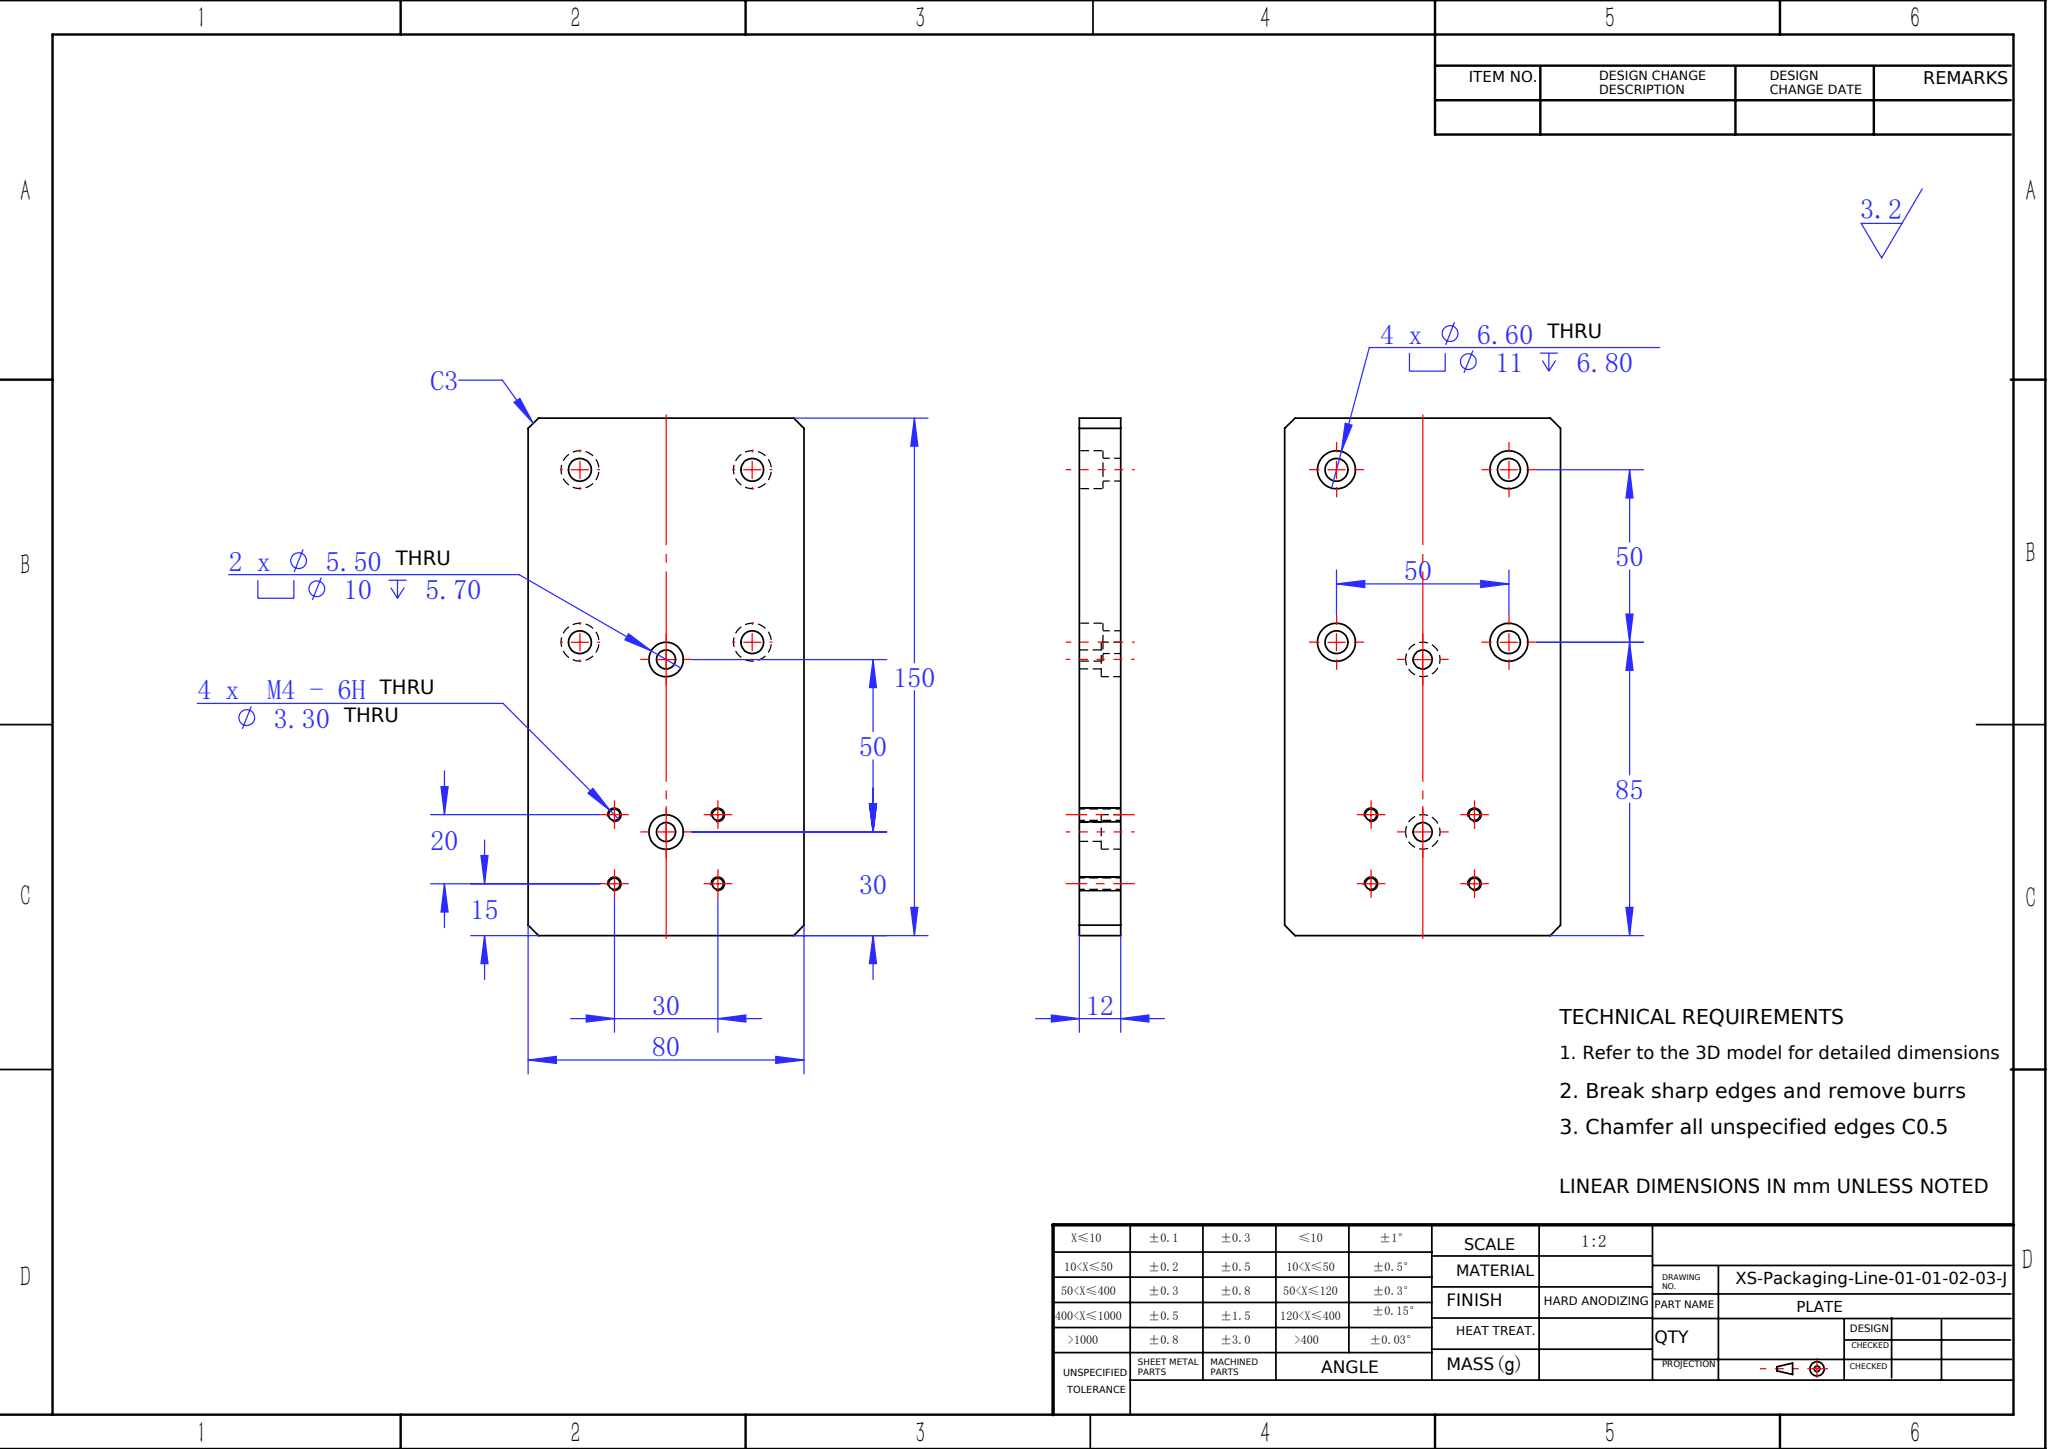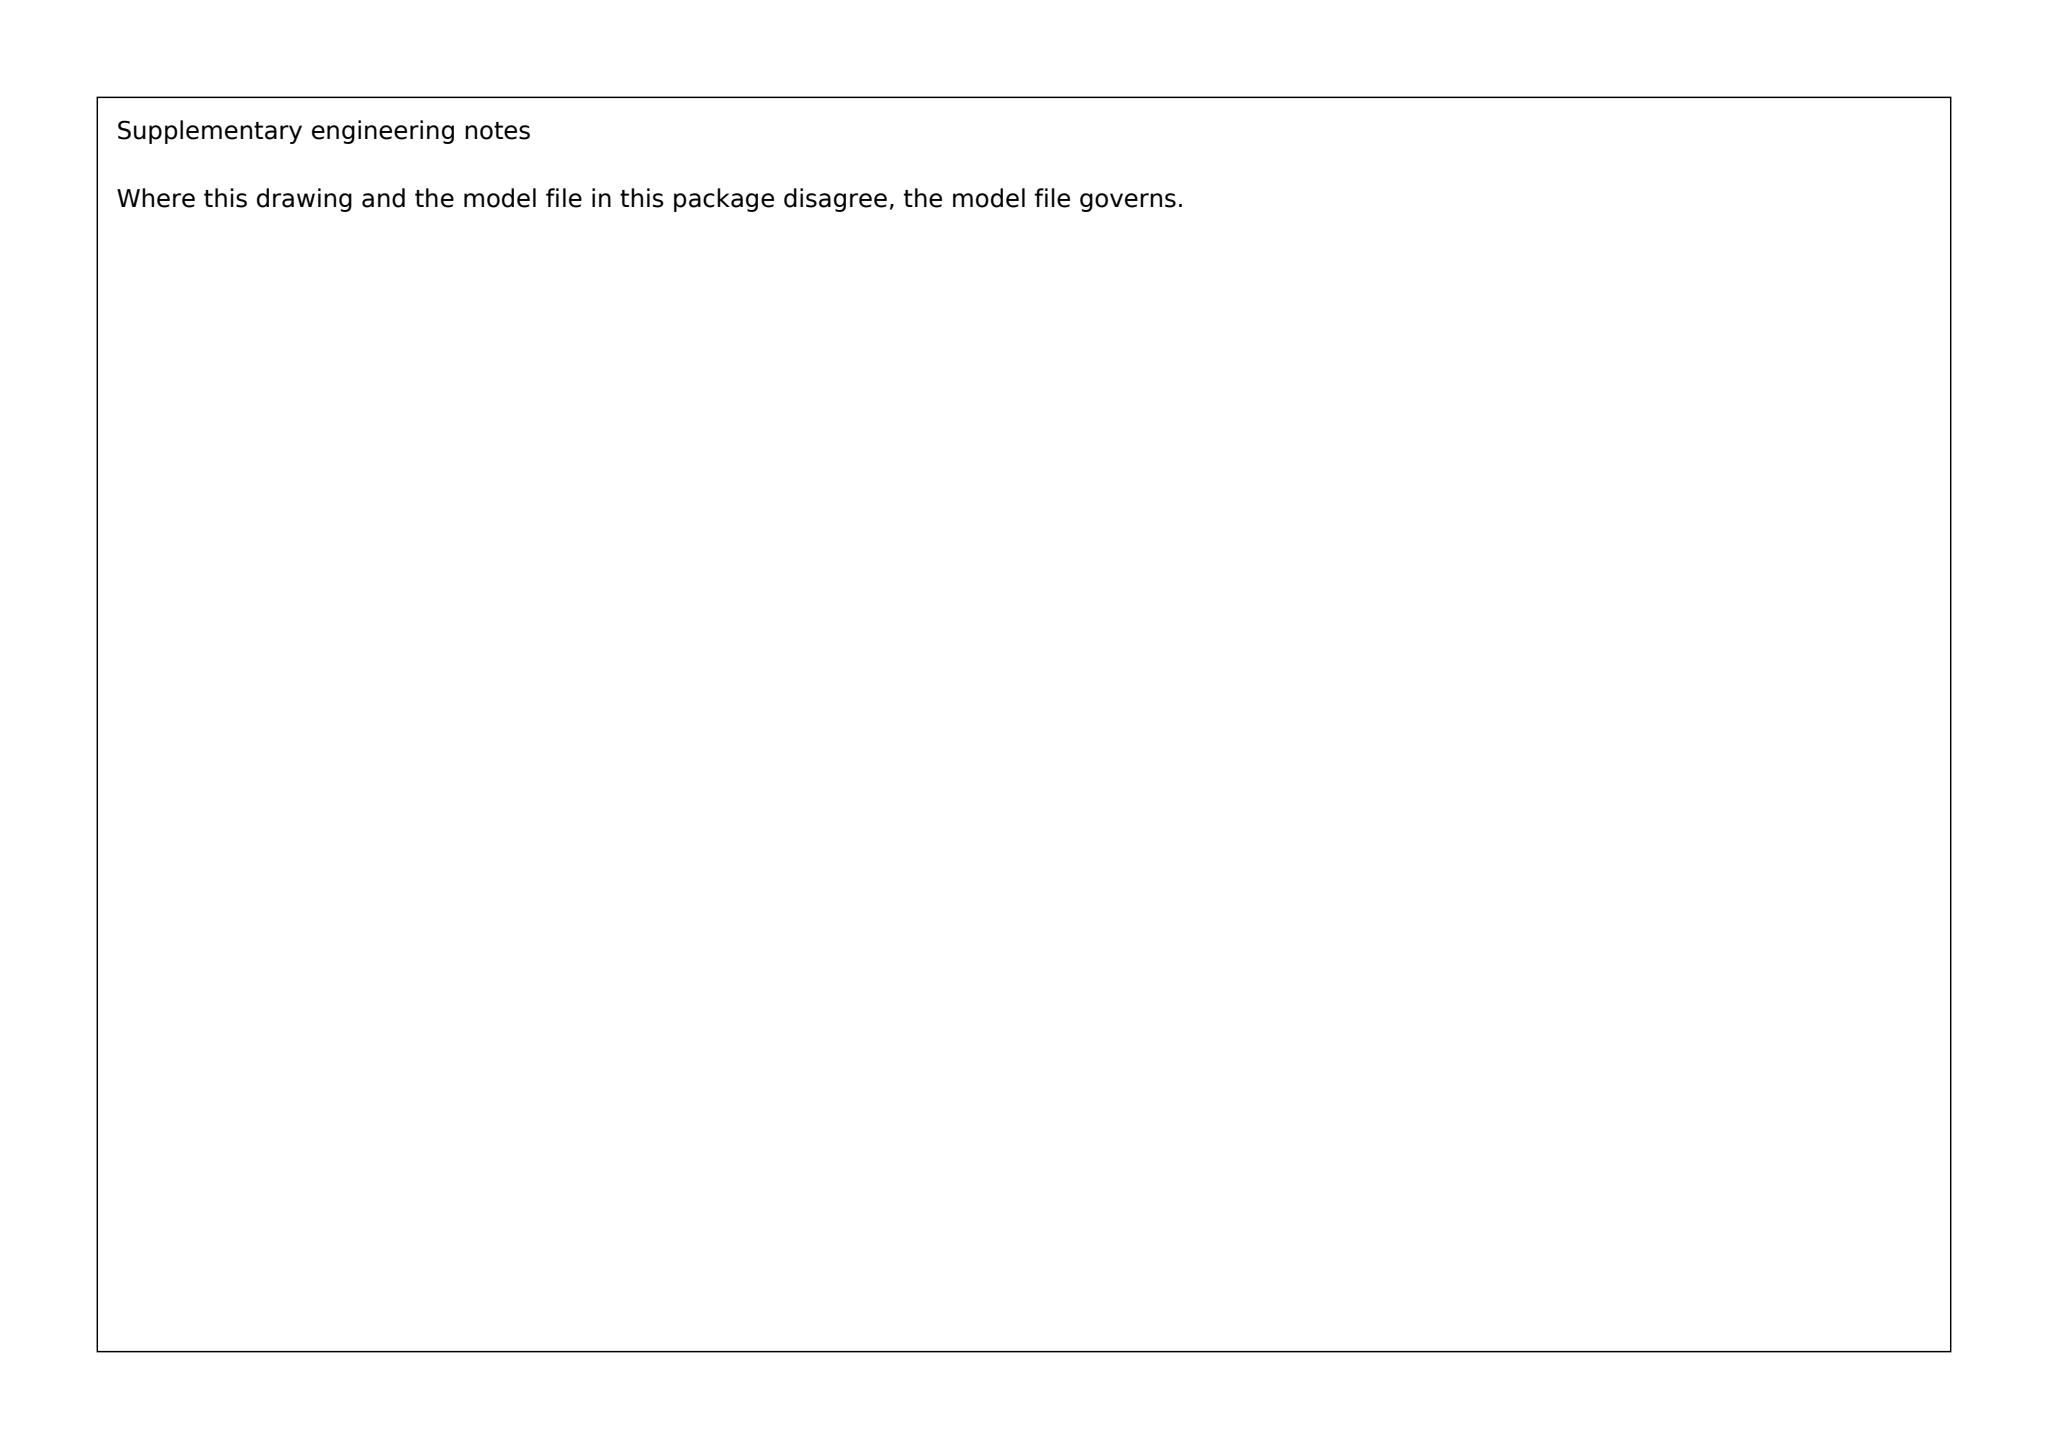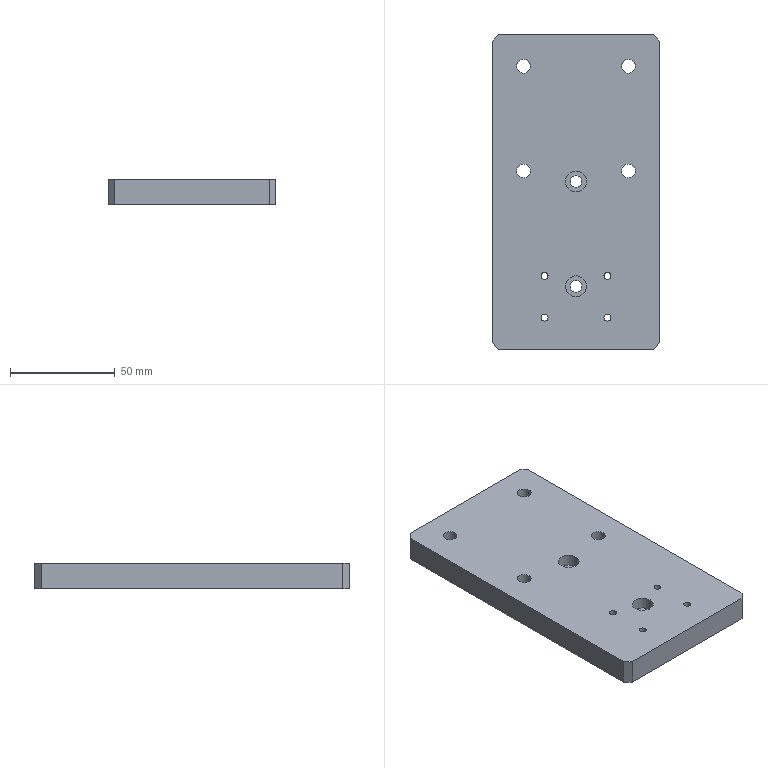Part | SolidWorks | mm | 1 solid | 48 faces | box 80 x 150 x 12 mm | volume 138882 mm3 | cylinder 32 | plane 16 | commonest cylinder face diameters 11 x8 6.6 x8 3.3 x8 10 x4 5.5 x4
build123d program:
from build123d import *

# Parameters (mm, degrees)
SKETCH1_W                                       = 80
SKETCH1_H                                       = 150
BOSS_EXTRUDE1_DEPTH                             = 12
CHAMFER1_SIZE                                   = 3
M4_TAPPED_HOLE1_D                               = 3.3
M6_HEX_SOCKET_HEAD_CAP_SCREW_CBORE1_D           = 6.6
M6_HEX_SOCKET_HEAD_CAP_SCREW_CBORE1_CBORE_D     = 11
M6_HEX_SOCKET_HEAD_CAP_SCREW_CBORE1_CBORE_DEPTH = 6.8
M5_HEX_SOCKET_HEAD_CAP_SCREW_CBORE1_D           = 5.5
M5_HEX_SOCKET_HEAD_CAP_SCREW_CBORE1_CBORE_D     = 10
M5_HEX_SOCKET_HEAD_CAP_SCREW_CBORE1_CBORE_DEPTH = 5.7


with BuildPart() as part:
    # Sketch1 → Boss-Extrude1 (new body)
    with BuildSketch(Plane.XY):
        Rectangle(SKETCH1_W, SKETCH1_H)
    extrude(amount=BOSS_EXTRUDE1_DEPTH)

    # Chamfer1
    chamfer1_edges = [part.edges().sort_by_distance(p)[0] for p in [
        (40, -75, 6),
        (-40, -75, 6),
        (-40, 75, 6),
        (40, 75, 6),
    ]]
    chamfer(chamfer1_edges, length=CHAMFER1_SIZE)

    # M4 Tapped Hole1 (through all)
    with Locations(Plane.XY.offset(12)):
        with Locations((-15, -40), (15, -40), (-15, -60), (15, -60)):
            Hole(M4_TAPPED_HOLE1_D / 2)

    # M6 Hex Socket Head Cap Screw CBORE1 (through all)
    with Locations(Plane(origin=(0, 0, 0), x_dir=(-1, 0, 0), z_dir=(0, 0, -1))):
        with Locations((-25, 60), (25, 60), (-25, 10), (25, 10)):
            CounterBoreHole(M6_HEX_SOCKET_HEAD_CAP_SCREW_CBORE1_D / 2, M6_HEX_SOCKET_HEAD_CAP_SCREW_CBORE1_CBORE_D / 2, M6_HEX_SOCKET_HEAD_CAP_SCREW_CBORE1_CBORE_DEPTH)

    # M5 Hex Socket Head Cap Screw CBORE1 (through all)
    with Locations(Plane.XY.offset(12)):
        with Locations((0, -45), (0, 5)):
            CounterBoreHole(M5_HEX_SOCKET_HEAD_CAP_SCREW_CBORE1_D / 2, M5_HEX_SOCKET_HEAD_CAP_SCREW_CBORE1_CBORE_D / 2, M5_HEX_SOCKET_HEAD_CAP_SCREW_CBORE1_CBORE_DEPTH)


solid = part.part